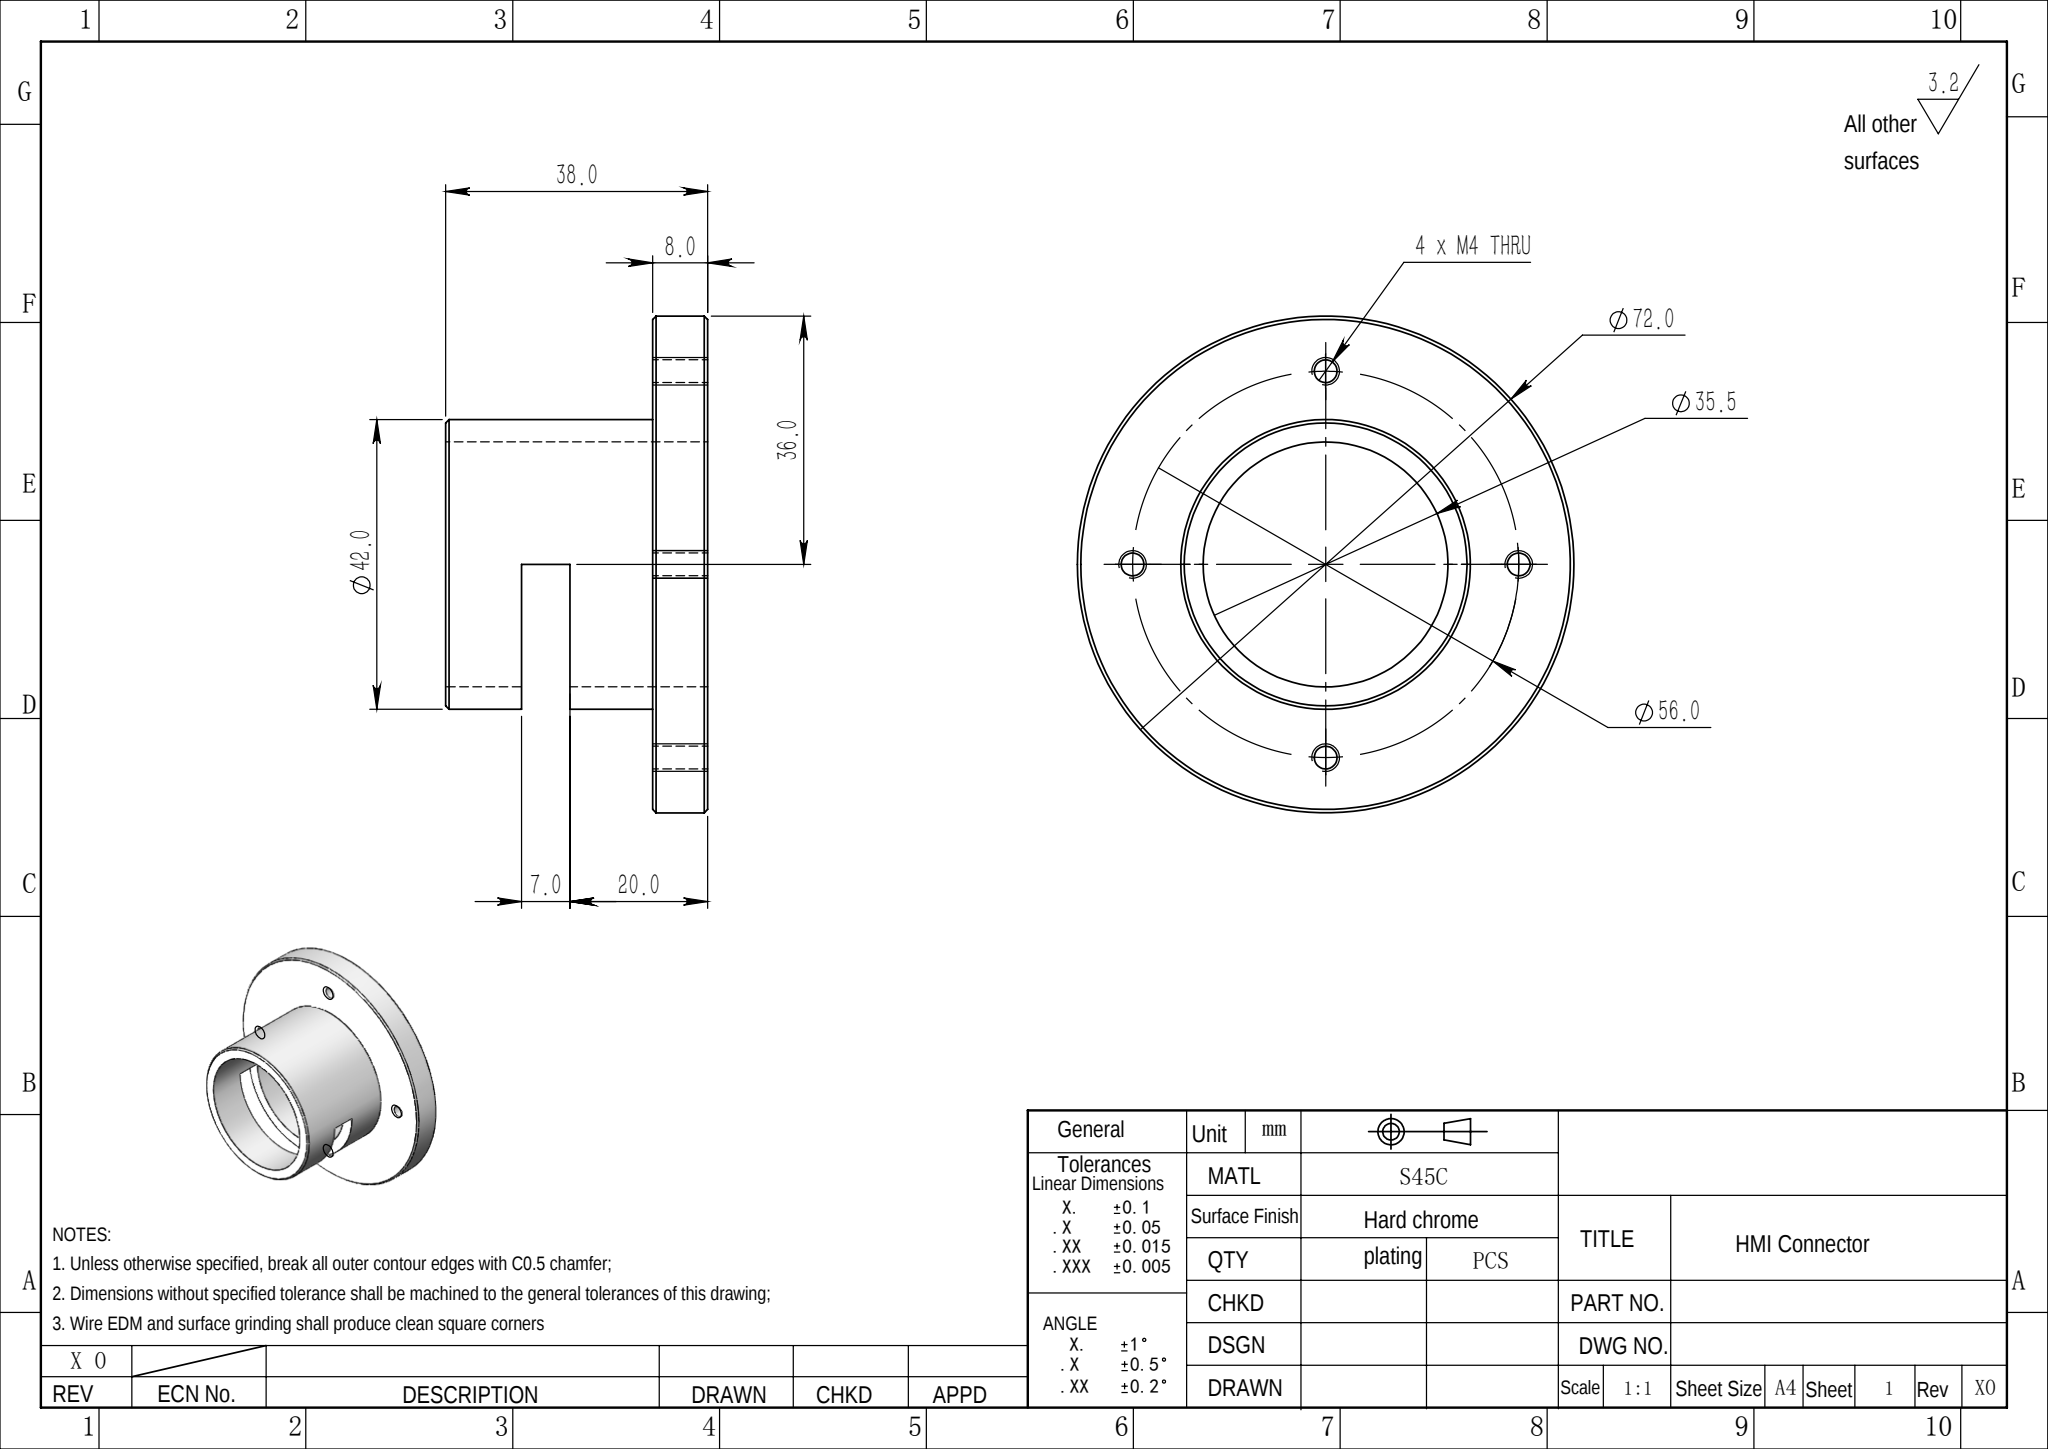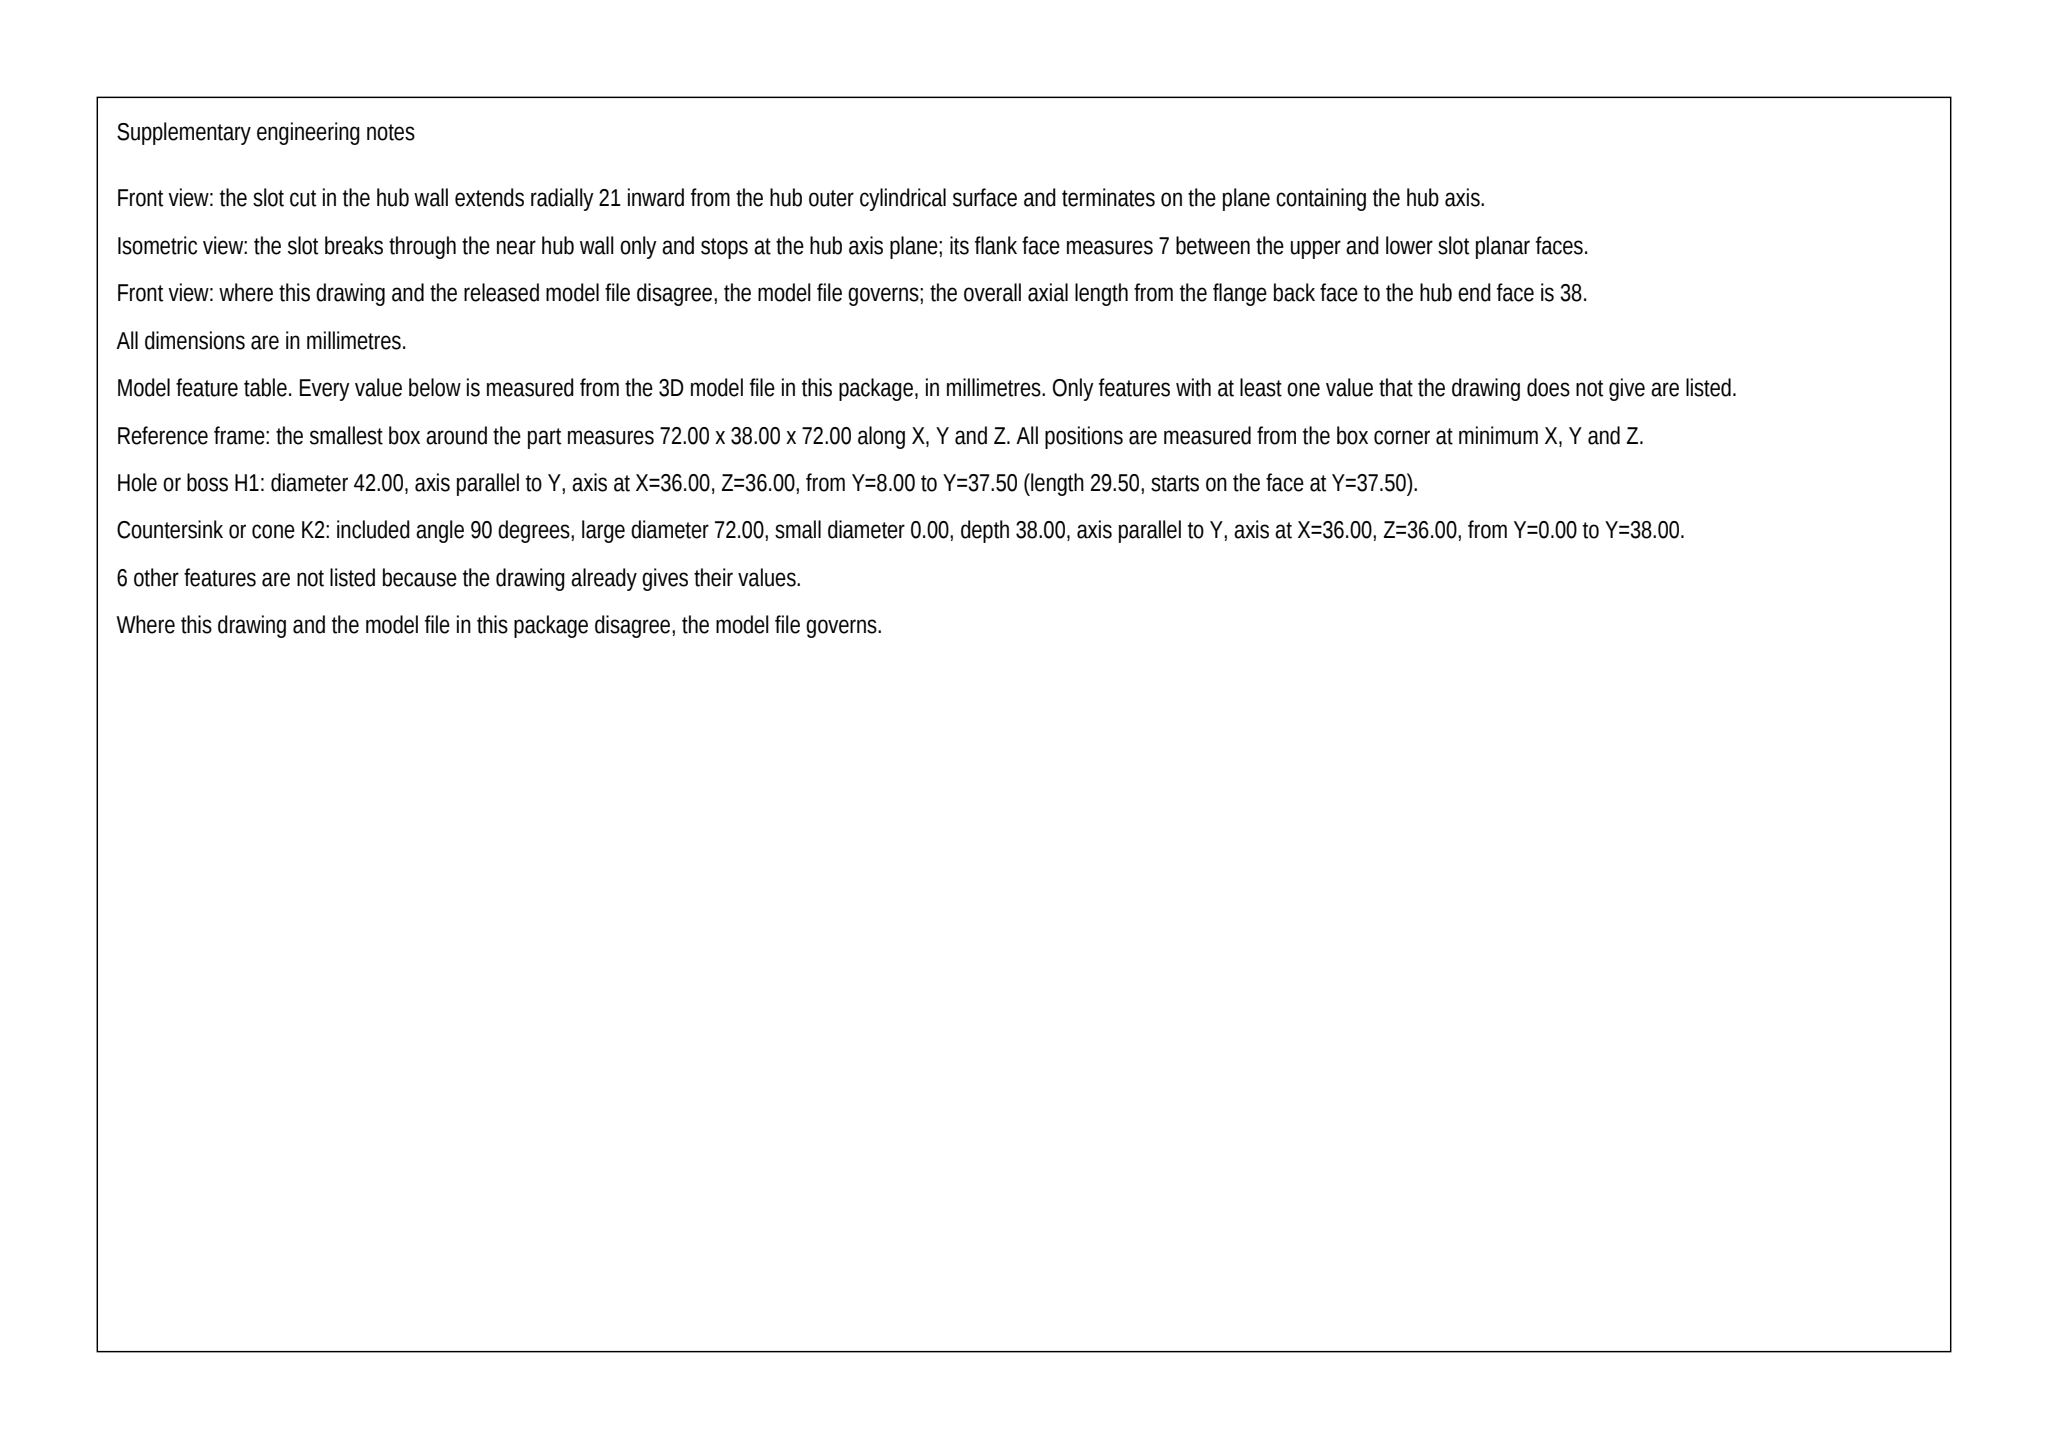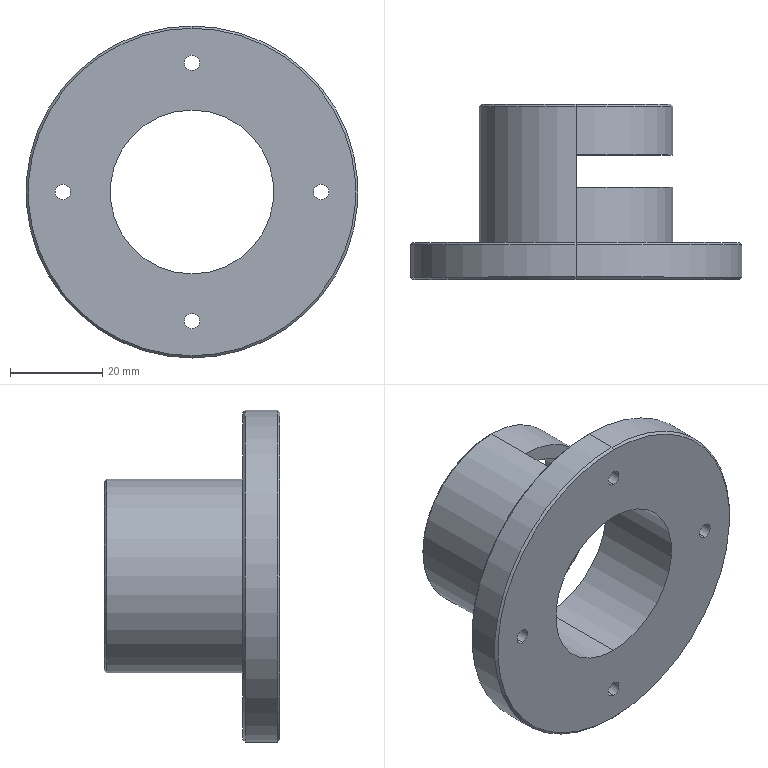Part | SolidWorks | mm | material S45C | 1 solid | 29 faces | box 72 x 38 x 72 mm | volume 34792 mm3 | cylinder 16 | plane 7 | cone 6 | commonest cylinder face diameters 3.3 x8 35.5 x3 42 x3 72 x2
build123d program:
from build123d import *

# Parameters (mm, degrees)
SKETCH1_R           = 36
BOSS_EXTRUDE1_DEPTH = 8
SKETCH2_R           = 21
BOSS_EXTRUDE2_DEPTH = 30
SKETCH3_R           = 17.75
CUT_EXTRUDE1_DEPTH  = 64.53
M4_TAPPED_HOLE1_D   = 3.3
CIRPATTERN1_COUNT   = 4
CHAMFER1_SIZE       = 0.5
CUT_EXTRUDE2_START  = -21
SKETCH6_W           = 45
SKETCH6_H           = 7
CUT_EXTRUDE2_DEPTH  = 21


with BuildPart() as part:
    # Sketch1 → Boss-Extrude1 (new body)
    with BuildSketch(Plane(origin=(0, 0, 0), x_dir=(1, 0, 0), z_dir=(0, 1, 0))):
        with Locations(Location((0, 0, 0), (0, 0, 270))):
            Circle(SKETCH1_R)
    extrude(amount=-BOSS_EXTRUDE1_DEPTH)

    # Sketch2 → Boss-Extrude2 (add)
    with BuildSketch(Plane(origin=(0, 0, 0), x_dir=(1, 0, 0), z_dir=(0, 1, 0))):
        with Locations(Location((0, 0, 0), (0, 0, 270))):
            Circle(SKETCH2_R)
    extrude(amount=BOSS_EXTRUDE2_DEPTH)

    # Sketch3 → Cut-Extrude1 (cut, through all)
    with BuildSketch(Plane(origin=(0, 30, 0), x_dir=(1, 0, 0), z_dir=(0, 1, 0))):
        with Locations(Location((0, 0, 0), (0, 0, 270))):
            Circle(SKETCH3_R)
    extrude(amount=-CUT_EXTRUDE1_DEPTH, mode=Mode.SUBTRACT)

    # M4 Tapped Hole1 (through all)
    with Locations(Plane(origin=(0, 0, 0), x_dir=(1, 0, 0), z_dir=(0, 1, 0))):
        with Locations((0, 28)):
            m4_tapped_hole1 = Hole(M4_TAPPED_HOLE1_D / 2)

    # CirPattern1: M4 Tapped Hole1 ×4 about axis
    cirpattern1_axis = Axis((0, 0, 0), (0, 1, 0))
    for i in range(1, CIRPATTERN1_COUNT):
        add(m4_tapped_hole1.rotate(cirpattern1_axis, i * 360 / CIRPATTERN1_COUNT), mode=Mode.SUBTRACT)

    # Chamfer1
    chamfer1_edges = [part.edges().sort_by_distance(p)[0] for p in [
        (0, 0, -36),
        (0, -8, -36),
        (0, 30, -21),
    ]]
    chamfer(chamfer1_edges, length=CHAMFER1_SIZE)

    # Sketch6 → Cut-Extrude2 (cut)
    with BuildSketch(Plane(origin=(21, 0, 0), x_dir=(0, 0, -1), z_dir=(1, 0, 0)).offset(CUT_EXTRUDE2_START)):
        with Locations((0, 15.5)):
            Rectangle(SKETCH6_W, SKETCH6_H)
    extrude(amount=CUT_EXTRUDE2_DEPTH, mode=Mode.SUBTRACT)


solid = part.part
STEP:
#1=CARTESIAN_POINT('',(0.,0.,35.5));
#2=VERTEX_POINT('',#1);
#3=CARTESIAN_POINT('',(0.,0.,-35.5));
#4=VERTEX_POINT('',#3);
#5=CARTESIAN_POINT('',(0.,0.,0.));
#6=DIRECTION('',(0.,1.,0.));
#7=DIRECTION('',(0.,0.,1.));
#8=AXIS2_PLACEMENT_3D('',#5,#6,#7);
#9=CIRCLE('',#8,35.5);
#10=EDGE_CURVE('',#2,#4,#9,.T.);
#11=ORIENTED_EDGE('',*,*,#10,.F.);
#12=CARTESIAN_POINT('',(0.,-0.5,36.));
#13=VERTEX_POINT('',#12);
#14=CARTESIAN_POINT('',(0.,0.,35.5));
#15=DIRECTION('',(0.,-0.7071,0.7071));
#16=VECTOR('',#15,1000.);
#17=LINE('',#14,#16);
#18=EDGE_CURVE('',#2,#13,#17,.T.);
#19=ORIENTED_EDGE('',*,*,#18,.T.);
#20=CARTESIAN_POINT('',(0.,-0.5,-36.));
#21=VERTEX_POINT('',#20);
#22=CARTESIAN_POINT('',(0.,-0.5,0.));
#23=DIRECTION('',(0.,-1.,0.));
#24=DIRECTION('',(0.,0.,1.));
#25=AXIS2_PLACEMENT_3D('',#22,#23,#24);
#26=CIRCLE('',#25,36.);
#27=EDGE_CURVE('',#21,#13,#26,.T.);
#28=ORIENTED_EDGE('',*,*,#27,.F.);
#29=CARTESIAN_POINT('',(0.,0.,-35.5));
#30=DIRECTION('',(0.,-0.7071,-0.7071));
#31=VECTOR('',#30,1000.);
#32=LINE('',#29,#31);
#33=EDGE_CURVE('',#4,#21,#32,.T.);
#34=ORIENTED_EDGE('',*,*,#33,.F.);
#35=EDGE_LOOP('',(#11,#19,#28,#34));
#36=FACE_OUTER_BOUND('',#35,.T.);
#37=CARTESIAN_POINT('',(0.,0.,0.));
#38=DIRECTION('',(0.,-1.,0.));
#39=DIRECTION('',(0.,0.,-1.));
#40=AXIS2_PLACEMENT_3D('',#37,#38,#39);
#41=CONICAL_SURFACE('',#40,35.5,0.7854);
#42=ADVANCED_FACE('',(#36),#41,.T.);
#43=CARTESIAN_POINT('',(0.,-8.,-35.5));
#44=VERTEX_POINT('',#43);
#45=CARTESIAN_POINT('',(0.,-8.,35.5));
#46=VERTEX_POINT('',#45);
#47=CARTESIAN_POINT('',(0.,-8.,0.));
#48=DIRECTION('',(0.,-1.,0.));
#49=DIRECTION('',(0.,0.,1.));
#50=AXIS2_PLACEMENT_3D('',#47,#48,#49);
#51=CIRCLE('',#50,35.5);
#52=EDGE_CURVE('',#44,#46,#51,.T.);
#53=ORIENTED_EDGE('',*,*,#52,.F.);
#54=CARTESIAN_POINT('',(0.,-7.5,-36.));
#55=VERTEX_POINT('',#54);
#56=CARTESIAN_POINT('',(0.,-7.5,-36.));
#57=DIRECTION('',(0.,0.7071,-0.7071));
#58=VECTOR('',#57,1000.);
#59=LINE('',#56,#58);
#60=EDGE_CURVE('',#44,#55,#59,.T.);
#61=ORIENTED_EDGE('',*,*,#60,.T.);
#62=CARTESIAN_POINT('',(0.,-7.5,36.));
#63=VERTEX_POINT('',#62);
#64=CARTESIAN_POINT('',(0.,-7.5,0.));
#65=DIRECTION('',(0.,1.,0.));
#66=DIRECTION('',(0.,0.,1.));
#67=AXIS2_PLACEMENT_3D('',#64,#65,#66);
#68=CIRCLE('',#67,36.);
#69=EDGE_CURVE('',#63,#55,#68,.T.);
#70=ORIENTED_EDGE('',*,*,#69,.F.);
#71=CARTESIAN_POINT('',(0.,-7.5,36.));
#72=DIRECTION('',(0.,0.7071,0.7071));
#73=VECTOR('',#72,1000.);
#74=LINE('',#71,#73);
#75=EDGE_CURVE('',#46,#63,#74,.T.);
#76=ORIENTED_EDGE('',*,*,#75,.F.);
#77=EDGE_LOOP('',(#53,#61,#70,#76));
#78=FACE_OUTER_BOUND('',#77,.T.);
#79=CARTESIAN_POINT('',(0.,-7.5,0.));
#80=DIRECTION('',(0.,1.,0.));
#81=DIRECTION('',(0.,0.,1.));
#82=AXIS2_PLACEMENT_3D('',#79,#80,#81);
#83=CONICAL_SURFACE('',#82,36.,0.7854);
#84=ADVANCED_FACE('',(#78),#83,.T.);
#85=CARTESIAN_POINT('',(0.,30.,20.5));
#86=VERTEX_POINT('',#85);
#87=CARTESIAN_POINT('',(0.,30.,-20.5));
#88=VERTEX_POINT('',#87);
#89=CARTESIAN_POINT('',(0.,30.,0.));
#90=DIRECTION('',(0.,1.,0.));
#91=DIRECTION('',(0.,0.,1.));
#92=AXIS2_PLACEMENT_3D('',#89,#90,#91);
#93=CIRCLE('',#92,20.5);
#94=EDGE_CURVE('',#86,#88,#93,.T.);
#95=ORIENTED_EDGE('',*,*,#94,.F.);
#96=CARTESIAN_POINT('',(0.,29.5,21.));
#97=VERTEX_POINT('',#96);
#98=CARTESIAN_POINT('',(0.,30.,20.5));
#99=DIRECTION('',(0.,-0.7071,0.7071));
#100=VECTOR('',#99,1000.);
#101=LINE('',#98,#100);
#102=EDGE_CURVE('',#86,#97,#101,.T.);
#103=ORIENTED_EDGE('',*,*,#102,.T.);
#104=CARTESIAN_POINT('',(0.,29.5,-21.));
#105=VERTEX_POINT('',#104);
#106=CARTESIAN_POINT('',(0.,29.5,0.));
#107=DIRECTION('',(0.,-1.,0.));
#108=DIRECTION('',(0.,0.,1.));
#109=AXIS2_PLACEMENT_3D('',#106,#107,#108);
#110=CIRCLE('',#109,21.);
#111=EDGE_CURVE('',#105,#97,#110,.T.);
#112=ORIENTED_EDGE('',*,*,#111,.F.);
#113=CARTESIAN_POINT('',(0.,30.,-20.5));
#114=DIRECTION('',(0.,-0.7071,-0.7071));
#115=VECTOR('',#114,1000.);
#116=LINE('',#113,#115);
#117=EDGE_CURVE('',#88,#105,#116,.T.);
#118=ORIENTED_EDGE('',*,*,#117,.F.);
#119=EDGE_LOOP('',(#95,#103,#112,#118));
#120=FACE_OUTER_BOUND('',#119,.T.);
#121=CARTESIAN_POINT('',(0.,30.,0.));
#122=DIRECTION('',(0.,-1.,0.));
#123=DIRECTION('',(0.,0.,-1.));
#124=AXIS2_PLACEMENT_3D('',#121,#122,#123);
#125=CONICAL_SURFACE('',#124,20.5,0.7854);
#126=ADVANCED_FACE('',(#120),#125,.T.);
#127=CARTESIAN_POINT('',(28.,-8.,-1.65));
#128=VERTEX_POINT('',#127);
#129=CARTESIAN_POINT('',(28.,-8.,1.65));
#130=VERTEX_POINT('',#129);
#131=CARTESIAN_POINT('',(28.,-8.,-0.));
#132=DIRECTION('',(0.,1.,0.));
#133=DIRECTION('',(0.,0.,1.));
#134=AXIS2_PLACEMENT_3D('',#131,#132,#133);
#135=CIRCLE('',#134,1.65);
#136=EDGE_CURVE('',#128,#130,#135,.T.);
#137=ORIENTED_EDGE('',*,*,#136,.F.);
#138=CARTESIAN_POINT('',(28.,0.,-1.65));
#139=VERTEX_POINT('',#138);
#140=CARTESIAN_POINT('',(28.,0.,-1.65));
#141=DIRECTION('',(0.,1.,0.));
#142=VECTOR('',#141,1000.);
#143=LINE('',#140,#142);
#144=EDGE_CURVE('',#128,#139,#143,.T.);
#145=ORIENTED_EDGE('',*,*,#144,.T.);
#146=CARTESIAN_POINT('',(28.,0.,1.65));
#147=VERTEX_POINT('',#146);
#148=CARTESIAN_POINT('',(28.,0.,-0.));
#149=DIRECTION('',(0.,1.,0.));
#150=DIRECTION('',(0.,0.,1.));
#151=AXIS2_PLACEMENT_3D('',#148,#149,#150);
#152=CIRCLE('',#151,1.65);
#153=EDGE_CURVE('',#139,#147,#152,.T.);
#154=ORIENTED_EDGE('',*,*,#153,.T.);
#155=CARTESIAN_POINT('',(28.,0.,1.65));
#156=DIRECTION('',(0.,1.,0.));
#157=VECTOR('',#156,1000.);
#158=LINE('',#155,#157);
#159=EDGE_CURVE('',#130,#147,#158,.T.);
#160=ORIENTED_EDGE('',*,*,#159,.F.);
#161=EDGE_LOOP('',(#137,#145,#154,#160));
#162=FACE_OUTER_BOUND('',#161,.T.);
#163=CARTESIAN_POINT('',(28.,0.,-0.));
#164=DIRECTION('',(0.,1.,0.));
#165=DIRECTION('',(0.,0.,1.));
#166=AXIS2_PLACEMENT_3D('',#163,#164,#165);
#167=CYLINDRICAL_SURFACE('',#166,1.65);
#168=ADVANCED_FACE('',(#162),#167,.F.);
#169=CARTESIAN_POINT('',(0.,-8.,26.35));
#170=VERTEX_POINT('',#169);
#171=CARTESIAN_POINT('',(0.,-8.,29.65));
#172=VERTEX_POINT('',#171);
#173=CARTESIAN_POINT('',(0.,-8.,28.));
#174=DIRECTION('',(0.,1.,0.));
#175=DIRECTION('',(0.,0.,1.));
#176=AXIS2_PLACEMENT_3D('',#173,#174,#175);
#177=CIRCLE('',#176,1.65);
#178=EDGE_CURVE('',#170,#172,#177,.T.);
#179=ORIENTED_EDGE('',*,*,#178,.F.);
#180=CARTESIAN_POINT('',(0.,0.,26.35));
#181=VERTEX_POINT('',#180);
#182=CARTESIAN_POINT('',(0.,0.,26.35));
#183=DIRECTION('',(0.,1.,0.));
#184=VECTOR('',#183,1000.);
#185=LINE('',#182,#184);
#186=EDGE_CURVE('',#170,#181,#185,.T.);
#187=ORIENTED_EDGE('',*,*,#186,.T.);
#188=CARTESIAN_POINT('',(0.,0.,29.65));
#189=VERTEX_POINT('',#188);
#190=CARTESIAN_POINT('',(0.,0.,28.));
#191=DIRECTION('',(0.,1.,0.));
#192=DIRECTION('',(0.,0.,1.));
#193=AXIS2_PLACEMENT_3D('',#190,#191,#192);
#194=CIRCLE('',#193,1.65);
#195=EDGE_CURVE('',#181,#189,#194,.T.);
#196=ORIENTED_EDGE('',*,*,#195,.T.);
#197=CARTESIAN_POINT('',(0.,0.,29.65));
#198=DIRECTION('',(0.,1.,0.));
#199=VECTOR('',#198,1000.);
#200=LINE('',#197,#199);
#201=EDGE_CURVE('',#172,#189,#200,.T.);
#202=ORIENTED_EDGE('',*,*,#201,.F.);
#203=EDGE_LOOP('',(#179,#187,#196,#202));
#204=FACE_OUTER_BOUND('',#203,.T.);
#205=CARTESIAN_POINT('',(0.,0.,28.));
#206=DIRECTION('',(0.,1.,0.));
#207=DIRECTION('',(0.,0.,1.));
#208=AXIS2_PLACEMENT_3D('',#205,#206,#207);
#209=CYLINDRICAL_SURFACE('',#208,1.65);
#210=ADVANCED_FACE('',(#204),#209,.F.);
#211=CARTESIAN_POINT('',(-28.,-8.,-1.65));
#212=VERTEX_POINT('',#211);
#213=CARTESIAN_POINT('',(-28.,-8.,1.65));
#214=VERTEX_POINT('',#213);
#215=CARTESIAN_POINT('',(-28.,-8.,0.));
#216=DIRECTION('',(0.,1.,0.));
#217=DIRECTION('',(0.,0.,1.));
#218=AXIS2_PLACEMENT_3D('',#215,#216,#217);
#219=CIRCLE('',#218,1.65);
#220=EDGE_CURVE('',#212,#214,#219,.T.);
#221=ORIENTED_EDGE('',*,*,#220,.F.);
#222=CARTESIAN_POINT('',(-28.,0.,-1.65));
#223=VERTEX_POINT('',#222);
#224=CARTESIAN_POINT('',(-28.,0.,-1.65));
#225=DIRECTION('',(0.,1.,0.));
#226=VECTOR('',#225,1000.);
#227=LINE('',#224,#226);
#228=EDGE_CURVE('',#212,#223,#227,.T.);
#229=ORIENTED_EDGE('',*,*,#228,.T.);
#230=CARTESIAN_POINT('',(-28.,0.,1.65));
#231=VERTEX_POINT('',#230);
#232=CARTESIAN_POINT('',(-28.,0.,0.));
#233=DIRECTION('',(0.,1.,0.));
#234=DIRECTION('',(0.,0.,1.));
#235=AXIS2_PLACEMENT_3D('',#232,#233,#234);
#236=CIRCLE('',#235,1.65);
#237=EDGE_CURVE('',#223,#231,#236,.T.);
#238=ORIENTED_EDGE('',*,*,#237,.T.);
#239=CARTESIAN_POINT('',(-28.,0.,1.65));
#240=DIRECTION('',(0.,1.,0.));
#241=VECTOR('',#240,1000.);
#242=LINE('',#239,#241);
#243=EDGE_CURVE('',#214,#231,#242,.T.);
#244=ORIENTED_EDGE('',*,*,#243,.F.);
#245=EDGE_LOOP('',(#221,#229,#238,#244));
#246=FACE_OUTER_BOUND('',#245,.T.);
#247=CARTESIAN_POINT('',(-28.,0.,0.));
#248=DIRECTION('',(0.,1.,0.));
#249=DIRECTION('',(0.,0.,1.));
#250=AXIS2_PLACEMENT_3D('',#247,#248,#249);
#251=CYLINDRICAL_SURFACE('',#250,1.65);
#252=ADVANCED_FACE('',(#246),#251,.F.);
#253=CARTESIAN_POINT('',(0.,-8.,-29.65));
#254=VERTEX_POINT('',#253);
#255=CARTESIAN_POINT('',(0.,-8.,-26.35));
#256=VERTEX_POINT('',#255);
#257=CARTESIAN_POINT('',(0.,-8.,-28.));
#258=DIRECTION('',(0.,1.,0.));
#259=DIRECTION('',(0.,0.,1.));
#260=AXIS2_PLACEMENT_3D('',#257,#258,#259);
#261=CIRCLE('',#260,1.65);
#262=EDGE_CURVE('',#254,#256,#261,.T.);
#263=ORIENTED_EDGE('',*,*,#262,.F.);
#264=CARTESIAN_POINT('',(0.,0.,-29.65));
#265=VERTEX_POINT('',#264);
#266=CARTESIAN_POINT('',(0.,0.,-29.65));
#267=DIRECTION('',(0.,1.,0.));
#268=VECTOR('',#267,1000.);
#269=LINE('',#266,#268);
#270=EDGE_CURVE('',#254,#265,#269,.T.);
#271=ORIENTED_EDGE('',*,*,#270,.T.);
#272=CARTESIAN_POINT('',(0.,0.,-26.35));
#273=VERTEX_POINT('',#272);
#274=CARTESIAN_POINT('',(0.,0.,-28.));
#275=DIRECTION('',(0.,1.,0.));
#276=DIRECTION('',(0.,0.,1.));
#277=AXIS2_PLACEMENT_3D('',#274,#275,#276);
#278=CIRCLE('',#277,1.65);
#279=EDGE_CURVE('',#265,#273,#278,.T.);
#280=ORIENTED_EDGE('',*,*,#279,.T.);
#281=CARTESIAN_POINT('',(0.,0.,-26.35));
#282=DIRECTION('',(0.,1.,0.));
#283=VECTOR('',#282,1000.);
#284=LINE('',#281,#283);
#285=EDGE_CURVE('',#256,#273,#284,.T.);
#286=ORIENTED_EDGE('',*,*,#285,.F.);
#287=EDGE_LOOP('',(#263,#271,#280,#286));
#288=FACE_OUTER_BOUND('',#287,.T.);
#289=CARTESIAN_POINT('',(0.,0.,-28.));
#290=DIRECTION('',(0.,1.,0.));
#291=DIRECTION('',(0.,0.,1.));
#292=AXIS2_PLACEMENT_3D('',#289,#290,#291);
#293=CYLINDRICAL_SURFACE('',#292,1.65);
#294=ADVANCED_FACE('',(#288),#293,.F.);
#295=ORIENTED_EDGE('',*,*,#69,.T.);
#296=CARTESIAN_POINT('',(0.,-8.,-36.));
#297=DIRECTION('',(0.,1.,0.));
#298=VECTOR('',#297,1000.);
#299=LINE('',#296,#298);
#300=EDGE_CURVE('',#55,#21,#299,.T.);
#301=ORIENTED_EDGE('',*,*,#300,.T.);
#302=ORIENTED_EDGE('',*,*,#27,.T.);
#303=CARTESIAN_POINT('',(0.,-8.,36.));
#304=DIRECTION('',(0.,1.,0.));
#305=VECTOR('',#304,1000.);
#306=LINE('',#303,#305);
#307=EDGE_CURVE('',#63,#13,#306,.T.);
#308=ORIENTED_EDGE('',*,*,#307,.F.);
#309=EDGE_LOOP('',(#295,#301,#302,#308));
#310=FACE_OUTER_BOUND('',#309,.T.);
#311=CARTESIAN_POINT('',(0.,-8.,0.));
#312=DIRECTION('',(0.,1.,0.));
#313=DIRECTION('',(0.,0.,1.));
#314=AXIS2_PLACEMENT_3D('',#311,#312,#313);
#315=CYLINDRICAL_SURFACE('',#314,36.);
#316=ADVANCED_FACE('',(#310),#315,.T.);
#317=CARTESIAN_POINT('',(0.,-8.,-17.75));
#318=VERTEX_POINT('',#317);
#319=CARTESIAN_POINT('',(0.,-8.,17.75));
#320=VERTEX_POINT('',#319);
#321=CARTESIAN_POINT('',(0.,-8.,0.));
#322=DIRECTION('',(0.,1.,0.));
#323=DIRECTION('',(0.,0.,1.));
#324=AXIS2_PLACEMENT_3D('',#321,#322,#323);
#325=CIRCLE('',#324,17.75);
#326=EDGE_CURVE('',#318,#320,#325,.T.);
#327=ORIENTED_EDGE('',*,*,#326,.F.);
#328=CARTESIAN_POINT('',(0.,12.,-17.75));
#329=VERTEX_POINT('',#328);
#330=CARTESIAN_POINT('',(0.,-8.,-17.75));
#331=DIRECTION('',(0.,1.,0.));
#332=VECTOR('',#331,1000.);
#333=LINE('',#330,#332);
#334=EDGE_CURVE('',#318,#329,#333,.T.);
#335=ORIENTED_EDGE('',*,*,#334,.T.);
#336=CARTESIAN_POINT('',(0.,19.,-17.75));
#337=VERTEX_POINT('',#336);
#338=CARTESIAN_POINT('',(0.,-8.,-17.75));
#339=DIRECTION('',(0.,-1.,0.));
#340=VECTOR('',#339,1000.);
#341=LINE('',#338,#340);
#342=EDGE_CURVE('',#337,#329,#341,.T.);
#343=ORIENTED_EDGE('',*,*,#342,.F.);
#344=CARTESIAN_POINT('',(0.,30.,-17.75));
#345=VERTEX_POINT('',#344);
#346=CARTESIAN_POINT('',(0.,-8.,-17.75));
#347=DIRECTION('',(0.,1.,0.));
#348=VECTOR('',#347,1000.);
#349=LINE('',#346,#348);
#350=EDGE_CURVE('',#337,#345,#349,.T.);
#351=ORIENTED_EDGE('',*,*,#350,.T.);
#352=CARTESIAN_POINT('',(0.,30.,17.75));
#353=VERTEX_POINT('',#352);
#354=CARTESIAN_POINT('',(0.,30.,0.));
#355=DIRECTION('',(0.,1.,0.));
#356=DIRECTION('',(0.,0.,1.));
#357=AXIS2_PLACEMENT_3D('',#354,#355,#356);
#358=CIRCLE('',#357,17.75);
#359=EDGE_CURVE('',#345,#353,#358,.T.);
#360=ORIENTED_EDGE('',*,*,#359,.T.);
#361=CARTESIAN_POINT('',(0.,19.,17.75));
#362=VERTEX_POINT('',#361);
#363=CARTESIAN_POINT('',(0.,-8.,17.75));
#364=DIRECTION('',(0.,1.,0.));
#365=VECTOR('',#364,1000.);
#366=LINE('',#363,#365);
#367=EDGE_CURVE('',#362,#353,#366,.T.);
#368=ORIENTED_EDGE('',*,*,#367,.F.);
#369=CARTESIAN_POINT('',(0.,12.,17.75));
#370=VERTEX_POINT('',#369);
#371=CARTESIAN_POINT('',(0.,-8.,17.75));
#372=DIRECTION('',(0.,1.,0.));
#373=VECTOR('',#372,1000.);
#374=LINE('',#371,#373);
#375=EDGE_CURVE('',#370,#362,#374,.T.);
#376=ORIENTED_EDGE('',*,*,#375,.F.);
#377=CARTESIAN_POINT('',(0.,-8.,17.75));
#378=DIRECTION('',(0.,1.,0.));
#379=VECTOR('',#378,1000.);
#380=LINE('',#377,#379);
#381=EDGE_CURVE('',#320,#370,#380,.T.);
#382=ORIENTED_EDGE('',*,*,#381,.F.);
#383=EDGE_LOOP('',(#327,#335,#343,#351,#360,#368,#376,#382));
#384=FACE_OUTER_BOUND('',#383,.T.);
#385=CARTESIAN_POINT('',(0.,-8.,0.));
#386=DIRECTION('',(0.,1.,0.));
#387=DIRECTION('',(0.,0.,1.));
#388=AXIS2_PLACEMENT_3D('',#385,#386,#387);
#389=CYLINDRICAL_SURFACE('',#388,17.75);
#390=ADVANCED_FACE('',(#384),#389,.F.);
#391=ORIENTED_EDGE('',*,*,#334,.F.);
#392=CARTESIAN_POINT('',(0.,-8.,0.));
#393=DIRECTION('',(0.,1.,0.));
#394=DIRECTION('',(0.,0.,1.));
#395=AXIS2_PLACEMENT_3D('',#392,#393,#394);
#396=CIRCLE('',#395,17.75);
#397=EDGE_CURVE('',#320,#318,#396,.T.);
#398=ORIENTED_EDGE('',*,*,#397,.F.);
#399=ORIENTED_EDGE('',*,*,#381,.T.);
#400=CARTESIAN_POINT('',(0.,12.,0.));
#401=DIRECTION('',(0.,1.,0.));
#402=DIRECTION('',(0.,0.,-1.));
#403=AXIS2_PLACEMENT_3D('',#400,#401,#402);
#404=CIRCLE('',#403,17.75);
#405=EDGE_CURVE('',#370,#329,#404,.T.);
#406=ORIENTED_EDGE('',*,*,#405,.T.);
#407=EDGE_LOOP('',(#391,#398,#399,#406));
#408=FACE_OUTER_BOUND('',#407,.T.);
#409=CARTESIAN_POINT('',(0.,-8.,0.));
#410=DIRECTION('',(0.,1.,0.));
#411=DIRECTION('',(0.,0.,1.));
#412=AXIS2_PLACEMENT_3D('',#409,#410,#411);
#413=CYLINDRICAL_SURFACE('',#412,17.75);
#414=ADVANCED_FACE('',(#408),#413,.F.);
#415=ORIENTED_EDGE('',*,*,#111,.T.);
#416=CARTESIAN_POINT('',(0.,19.,21.));
#417=VERTEX_POINT('',#416);
#418=CARTESIAN_POINT('',(0.,30.,21.));
#419=DIRECTION('',(0.,-1.,0.));
#420=VECTOR('',#419,1000.);
#421=LINE('',#418,#420);
#422=EDGE_CURVE('',#97,#417,#421,.T.);
#423=ORIENTED_EDGE('',*,*,#422,.T.);
#424=CARTESIAN_POINT('',(0.,19.,-21.));
#425=VERTEX_POINT('',#424);
#426=CARTESIAN_POINT('',(0.,19.,0.));
#427=DIRECTION('',(0.,1.,0.));
#428=DIRECTION('',(0.,0.,1.));
#429=AXIS2_PLACEMENT_3D('',#426,#427,#428);
#430=CIRCLE('',#429,21.);
#431=EDGE_CURVE('',#417,#425,#430,.T.);
#432=ORIENTED_EDGE('',*,*,#431,.T.);
#433=CARTESIAN_POINT('',(0.,30.,-21.));
#434=DIRECTION('',(0.,-1.,0.));
#435=VECTOR('',#434,1000.);
#436=LINE('',#433,#435);
#437=EDGE_CURVE('',#105,#425,#436,.T.);
#438=ORIENTED_EDGE('',*,*,#437,.F.);
#439=EDGE_LOOP('',(#415,#423,#432,#438));
#440=FACE_OUTER_BOUND('',#439,.T.);
#441=CARTESIAN_POINT('',(0.,30.,0.));
#442=DIRECTION('',(0.,-1.,0.));
#443=DIRECTION('',(0.,0.,-1.));
#444=AXIS2_PLACEMENT_3D('',#441,#442,#443);
#445=CYLINDRICAL_SURFACE('',#444,21.);
#446=ADVANCED_FACE('',(#440),#445,.T.);
#447=CARTESIAN_POINT('',(0.,12.,-21.));
#448=VERTEX_POINT('',#447);
#449=CARTESIAN_POINT('',(0.,12.,21.));
#450=VERTEX_POINT('',#449);
#451=CARTESIAN_POINT('',(0.,12.,0.));
#452=DIRECTION('',(0.,-1.,-0.));
#453=DIRECTION('',(0.,0.,-1.));
#454=AXIS2_PLACEMENT_3D('',#451,#452,#453);
#455=CIRCLE('',#454,21.);
#456=EDGE_CURVE('',#448,#450,#455,.T.);
#457=ORIENTED_EDGE('',*,*,#456,.T.);
#458=CARTESIAN_POINT('',(0.,0.,21.));
#459=VERTEX_POINT('',#458);
#460=CARTESIAN_POINT('',(0.,30.,21.));
#461=DIRECTION('',(0.,-1.,0.));
#462=VECTOR('',#461,1000.);
#463=LINE('',#460,#462);
#464=EDGE_CURVE('',#450,#459,#463,.T.);
#465=ORIENTED_EDGE('',*,*,#464,.T.);
#466=CARTESIAN_POINT('',(0.,0.,-21.));
#467=VERTEX_POINT('',#466);
#468=CARTESIAN_POINT('',(0.,0.,0.));
#469=DIRECTION('',(0.,1.,0.));
#470=DIRECTION('',(0.,0.,1.));
#471=AXIS2_PLACEMENT_3D('',#468,#469,#470);
#472=CIRCLE('',#471,21.);
#473=EDGE_CURVE('',#459,#467,#472,.T.);
#474=ORIENTED_EDGE('',*,*,#473,.T.);
#475=CARTESIAN_POINT('',(0.,30.,-21.));
#476=DIRECTION('',(0.,-1.,0.));
#477=VECTOR('',#476,1000.);
#478=LINE('',#475,#477);
#479=EDGE_CURVE('',#448,#467,#478,.T.);
#480=ORIENTED_EDGE('',*,*,#479,.F.);
#481=EDGE_LOOP('',(#457,#465,#474,#480));
#482=FACE_OUTER_BOUND('',#481,.T.);
#483=CARTESIAN_POINT('',(0.,30.,0.));
#484=DIRECTION('',(0.,-1.,0.));
#485=DIRECTION('',(0.,0.,-1.));
#486=AXIS2_PLACEMENT_3D('',#483,#484,#485);
#487=CYLINDRICAL_SURFACE('',#486,21.);
#488=ADVANCED_FACE('',(#482),#487,.T.);
#489=ORIENTED_EDGE('',*,*,#422,.F.);
#490=CARTESIAN_POINT('',(0.,29.5,0.));
#491=DIRECTION('',(0.,-1.,0.));
#492=DIRECTION('',(0.,0.,1.));
#493=AXIS2_PLACEMENT_3D('',#490,#491,#492);
#494=CIRCLE('',#493,21.);
#495=EDGE_CURVE('',#97,#105,#494,.T.);
#496=ORIENTED_EDGE('',*,*,#495,.T.);
#497=ORIENTED_EDGE('',*,*,#437,.T.);
#498=CARTESIAN_POINT('',(0.,30.,-21.));
#499=DIRECTION('',(0.,1.,0.));
#500=VECTOR('',#499,1000.);
#501=LINE('',#498,#500);
#502=EDGE_CURVE('',#448,#425,#501,.T.);
#503=ORIENTED_EDGE('',*,*,#502,.F.);
#504=ORIENTED_EDGE('',*,*,#479,.T.);
#505=CARTESIAN_POINT('',(0.,0.,0.));
#506=DIRECTION('',(0.,1.,0.));
#507=DIRECTION('',(0.,0.,1.));
#508=AXIS2_PLACEMENT_3D('',#505,#506,#507);
#509=CIRCLE('',#508,21.);
#510=EDGE_CURVE('',#467,#459,#509,.T.);
#511=ORIENTED_EDGE('',*,*,#510,.T.);
#512=ORIENTED_EDGE('',*,*,#464,.F.);
#513=CARTESIAN_POINT('',(0.,30.,21.));
#514=DIRECTION('',(0.,-1.,0.));
#515=VECTOR('',#514,1000.);
#516=LINE('',#513,#515);
#517=EDGE_CURVE('',#417,#450,#516,.T.);
#518=ORIENTED_EDGE('',*,*,#517,.F.);
#519=EDGE_LOOP('',(#489,#496,#497,#503,#504,#511,#512,#518));
#520=FACE_OUTER_BOUND('',#519,.T.);
#521=CARTESIAN_POINT('',(0.,30.,0.));
#522=DIRECTION('',(0.,-1.,0.));
#523=DIRECTION('',(0.,0.,-1.));
#524=AXIS2_PLACEMENT_3D('',#521,#522,#523);
#525=CYLINDRICAL_SURFACE('',#524,21.);
#526=ADVANCED_FACE('',(#520),#525,.T.);
#527=ORIENTED_EDGE('',*,*,#350,.F.);
#528=CARTESIAN_POINT('',(0.,19.,0.));
#529=DIRECTION('',(0.,-1.,0.));
#530=DIRECTION('',(0.,0.,1.));
#531=AXIS2_PLACEMENT_3D('',#528,#529,#530);
#532=CIRCLE('',#531,17.75);
#533=EDGE_CURVE('',#337,#362,#532,.T.);
#534=ORIENTED_EDGE('',*,*,#533,.T.);
#535=ORIENTED_EDGE('',*,*,#367,.T.);
#536=CARTESIAN_POINT('',(0.,30.,0.));
#537=DIRECTION('',(0.,1.,0.));
#538=DIRECTION('',(0.,0.,1.));
#539=AXIS2_PLACEMENT_3D('',#536,#537,#538);
#540=CIRCLE('',#539,17.75);
#541=EDGE_CURVE('',#353,#345,#540,.T.);
#542=ORIENTED_EDGE('',*,*,#541,.T.);
#543=EDGE_LOOP('',(#527,#534,#535,#542));
#544=FACE_OUTER_BOUND('',#543,.T.);
#545=CARTESIAN_POINT('',(0.,-8.,0.));
#546=DIRECTION('',(0.,1.,0.));
#547=DIRECTION('',(0.,0.,1.));
#548=AXIS2_PLACEMENT_3D('',#545,#546,#547);
#549=CYLINDRICAL_SURFACE('',#548,17.75);
#550=ADVANCED_FACE('',(#544),#549,.F.);
#551=ORIENTED_EDGE('',*,*,#300,.F.);
#552=CARTESIAN_POINT('',(0.,-7.5,0.));
#553=DIRECTION('',(0.,1.,0.));
#554=DIRECTION('',(0.,0.,1.));
#555=AXIS2_PLACEMENT_3D('',#552,#553,#554);
#556=CIRCLE('',#555,36.);
#557=EDGE_CURVE('',#55,#63,#556,.T.);
#558=ORIENTED_EDGE('',*,*,#557,.T.);
#559=ORIENTED_EDGE('',*,*,#307,.T.);
#560=CARTESIAN_POINT('',(0.,-0.5,0.));
#561=DIRECTION('',(0.,-1.,0.));
#562=DIRECTION('',(0.,0.,1.));
#563=AXIS2_PLACEMENT_3D('',#560,#561,#562);
#564=CIRCLE('',#563,36.);
#565=EDGE_CURVE('',#13,#21,#564,.T.);
#566=ORIENTED_EDGE('',*,*,#565,.T.);
#567=EDGE_LOOP('',(#551,#558,#559,#566));
#568=FACE_OUTER_BOUND('',#567,.T.);
#569=CARTESIAN_POINT('',(0.,-8.,0.));
#570=DIRECTION('',(0.,1.,0.));
#571=DIRECTION('',(0.,0.,1.));
#572=AXIS2_PLACEMENT_3D('',#569,#570,#571);
#573=CYLINDRICAL_SURFACE('',#572,36.);
#574=ADVANCED_FACE('',(#568),#573,.T.);
#575=CARTESIAN_POINT('',(0.,-8.,0.));
#576=DIRECTION('',(0.,-1.,0.));
#577=DIRECTION('',(0.,0.,1.));
#578=AXIS2_PLACEMENT_3D('',#575,#576,#577);
#579=CIRCLE('',#578,35.5);
#580=EDGE_CURVE('',#46,#44,#579,.T.);
#581=ORIENTED_EDGE('',*,*,#580,.T.);
#582=ORIENTED_EDGE('',*,*,#52,.T.);
#583=EDGE_LOOP('',(#581,#582));
#584=FACE_OUTER_BOUND('',#583,.T.);
#585=CARTESIAN_POINT('',(28.,-8.,-0.));
#586=DIRECTION('',(0.,1.,0.));
#587=DIRECTION('',(0.,0.,1.));
#588=AXIS2_PLACEMENT_3D('',#585,#586,#587);
#589=CIRCLE('',#588,1.65);
#590=EDGE_CURVE('',#130,#128,#589,.T.);
#591=ORIENTED_EDGE('',*,*,#590,.T.);
#592=ORIENTED_EDGE('',*,*,#136,.T.);
#593=EDGE_LOOP('',(#591,#592));
#594=FACE_BOUND('',#593,.T.);
#595=CARTESIAN_POINT('',(0.,-8.,28.));
#596=DIRECTION('',(0.,1.,0.));
#597=DIRECTION('',(0.,0.,1.));
#598=AXIS2_PLACEMENT_3D('',#595,#596,#597);
#599=CIRCLE('',#598,1.65);
#600=EDGE_CURVE('',#172,#170,#599,.T.);
#601=ORIENTED_EDGE('',*,*,#600,.T.);
#602=ORIENTED_EDGE('',*,*,#178,.T.);
#603=EDGE_LOOP('',(#601,#602));
#604=FACE_BOUND('',#603,.T.);
#605=CARTESIAN_POINT('',(-28.,-8.,0.));
#606=DIRECTION('',(0.,1.,0.));
#607=DIRECTION('',(0.,0.,1.));
#608=AXIS2_PLACEMENT_3D('',#605,#606,#607);
#609=CIRCLE('',#608,1.65);
#610=EDGE_CURVE('',#214,#212,#609,.T.);
#611=ORIENTED_EDGE('',*,*,#610,.T.);
#612=ORIENTED_EDGE('',*,*,#220,.T.);
#613=EDGE_LOOP('',(#611,#612));
#614=FACE_BOUND('',#613,.T.);
#615=CARTESIAN_POINT('',(0.,-8.,-28.));
#616=DIRECTION('',(0.,1.,0.));
#617=DIRECTION('',(0.,0.,1.));
#618=AXIS2_PLACEMENT_3D('',#615,#616,#617);
#619=CIRCLE('',#618,1.65);
#620=EDGE_CURVE('',#256,#254,#619,.T.);
#621=ORIENTED_EDGE('',*,*,#620,.T.);
#622=ORIENTED_EDGE('',*,*,#262,.T.);
#623=EDGE_LOOP('',(#621,#622));
#624=FACE_BOUND('',#623,.T.);
#625=ORIENTED_EDGE('',*,*,#397,.T.);
#626=ORIENTED_EDGE('',*,*,#326,.T.);
#627=EDGE_LOOP('',(#625,#626));
#628=FACE_BOUND('',#627,.T.);
#629=CARTESIAN_POINT('',(0.,-8.,0.));
#630=DIRECTION('',(0.,1.,0.));
#631=DIRECTION('',(0.,0.,1.));
#632=AXIS2_PLACEMENT_3D('',#629,#630,#631);
#633=PLANE('',#632);
#634=ADVANCED_FACE('',(#584,#594,#604,#614,#624,#628),#633,.F.);
#635=CARTESIAN_POINT('',(0.,0.,0.));
#636=DIRECTION('',(0.,1.,0.));
#637=DIRECTION('',(0.,0.,1.));
#638=AXIS2_PLACEMENT_3D('',#635,#636,#637);
#639=CIRCLE('',#638,35.5);
#640=EDGE_CURVE('',#4,#2,#639,.T.);
#641=ORIENTED_EDGE('',*,*,#640,.T.);
#642=ORIENTED_EDGE('',*,*,#10,.T.);
#643=EDGE_LOOP('',(#641,#642));
#644=FACE_OUTER_BOUND('',#643,.T.);
#645=CARTESIAN_POINT('',(28.,0.,-0.));
#646=DIRECTION('',(0.,1.,0.));
#647=DIRECTION('',(0.,0.,1.));
#648=AXIS2_PLACEMENT_3D('',#645,#646,#647);
#649=CIRCLE('',#648,1.65);
#650=EDGE_CURVE('',#147,#139,#649,.T.);
#651=ORIENTED_EDGE('',*,*,#650,.F.);
#652=ORIENTED_EDGE('',*,*,#153,.F.);
#653=EDGE_LOOP('',(#651,#652));
#654=FACE_BOUND('',#653,.T.);
#655=CARTESIAN_POINT('',(0.,0.,28.));
#656=DIRECTION('',(0.,1.,0.));
#657=DIRECTION('',(0.,0.,1.));
#658=AXIS2_PLACEMENT_3D('',#655,#656,#657);
#659=CIRCLE('',#658,1.65);
#660=EDGE_CURVE('',#189,#181,#659,.T.);
#661=ORIENTED_EDGE('',*,*,#660,.F.);
#662=ORIENTED_EDGE('',*,*,#195,.F.);
#663=EDGE_LOOP('',(#661,#662));
#664=FACE_BOUND('',#663,.T.);
#665=CARTESIAN_POINT('',(-28.,0.,0.));
#666=DIRECTION('',(0.,1.,0.));
#667=DIRECTION('',(0.,0.,1.));
#668=AXIS2_PLACEMENT_3D('',#665,#666,#667);
#669=CIRCLE('',#668,1.65);
#670=EDGE_CURVE('',#231,#223,#669,.T.);
#671=ORIENTED_EDGE('',*,*,#670,.F.);
#672=ORIENTED_EDGE('',*,*,#237,.F.);
#673=EDGE_LOOP('',(#671,#672));
#674=FACE_BOUND('',#673,.T.);
#675=CARTESIAN_POINT('',(0.,0.,-28.));
#676=DIRECTION('',(0.,1.,0.));
#677=DIRECTION('',(0.,0.,1.));
#678=AXIS2_PLACEMENT_3D('',#675,#676,#677);
#679=CIRCLE('',#678,1.65);
#680=EDGE_CURVE('',#273,#265,#679,.T.);
#681=ORIENTED_EDGE('',*,*,#680,.F.);
#682=ORIENTED_EDGE('',*,*,#279,.F.);
#683=EDGE_LOOP('',(#681,#682));
#684=FACE_BOUND('',#683,.T.);
#685=ORIENTED_EDGE('',*,*,#510,.F.);
#686=ORIENTED_EDGE('',*,*,#473,.F.);
#687=EDGE_LOOP('',(#685,#686));
#688=FACE_BOUND('',#687,.T.);
#689=CARTESIAN_POINT('',(0.,0.,0.));
#690=DIRECTION('',(0.,1.,0.));
#691=DIRECTION('',(0.,0.,1.));
#692=AXIS2_PLACEMENT_3D('',#689,#690,#691);
#693=PLANE('',#692);
#694=ADVANCED_FACE('',(#644,#654,#664,#674,#684,#688),#693,.T.);
#695=CARTESIAN_POINT('',(0.,30.,0.));
#696=DIRECTION('',(0.,1.,0.));
#697=DIRECTION('',(0.,0.,1.));
#698=AXIS2_PLACEMENT_3D('',#695,#696,#697);
#699=CIRCLE('',#698,20.5);
#700=EDGE_CURVE('',#88,#86,#699,.T.);
#701=ORIENTED_EDGE('',*,*,#700,.T.);
#702=ORIENTED_EDGE('',*,*,#94,.T.);
#703=EDGE_LOOP('',(#701,#702));
#704=FACE_OUTER_BOUND('',#703,.T.);
#705=ORIENTED_EDGE('',*,*,#541,.F.);
#706=ORIENTED_EDGE('',*,*,#359,.F.);
#707=EDGE_LOOP('',(#705,#706));
#708=FACE_BOUND('',#707,.T.);
#709=CARTESIAN_POINT('',(0.,30.,0.));
#710=DIRECTION('',(0.,1.,0.));
#711=DIRECTION('',(0.,0.,1.));
#712=AXIS2_PLACEMENT_3D('',#709,#710,#711);
#713=PLANE('',#712);
#714=ADVANCED_FACE('',(#704,#708),#713,.T.);
#715=ORIENTED_EDGE('',*,*,#270,.F.);
#716=ORIENTED_EDGE('',*,*,#620,.F.);
#717=ORIENTED_EDGE('',*,*,#285,.T.);
#718=ORIENTED_EDGE('',*,*,#680,.T.);
#719=EDGE_LOOP('',(#715,#716,#717,#718));
#720=FACE_OUTER_BOUND('',#719,.T.);
#721=CARTESIAN_POINT('',(0.,0.,-28.));
#722=DIRECTION('',(0.,1.,0.));
#723=DIRECTION('',(0.,0.,1.));
#724=AXIS2_PLACEMENT_3D('',#721,#722,#723);
#725=CYLINDRICAL_SURFACE('',#724,1.65);
#726=ADVANCED_FACE('',(#720),#725,.F.);
#727=ORIENTED_EDGE('',*,*,#228,.F.);
#728=ORIENTED_EDGE('',*,*,#610,.F.);
#729=ORIENTED_EDGE('',*,*,#243,.T.);
#730=ORIENTED_EDGE('',*,*,#670,.T.);
#731=EDGE_LOOP('',(#727,#728,#729,#730));
#732=FACE_OUTER_BOUND('',#731,.T.);
#733=CARTESIAN_POINT('',(-28.,0.,0.));
#734=DIRECTION('',(0.,1.,0.));
#735=DIRECTION('',(0.,0.,1.));
#736=AXIS2_PLACEMENT_3D('',#733,#734,#735);
#737=CYLINDRICAL_SURFACE('',#736,1.65);
#738=ADVANCED_FACE('',(#732),#737,.F.);
#739=ORIENTED_EDGE('',*,*,#186,.F.);
#740=ORIENTED_EDGE('',*,*,#600,.F.);
#741=ORIENTED_EDGE('',*,*,#201,.T.);
#742=ORIENTED_EDGE('',*,*,#660,.T.);
#743=EDGE_LOOP('',(#739,#740,#741,#742));
#744=FACE_OUTER_BOUND('',#743,.T.);
#745=CARTESIAN_POINT('',(0.,0.,28.));
#746=DIRECTION('',(0.,1.,0.));
#747=DIRECTION('',(0.,0.,1.));
#748=AXIS2_PLACEMENT_3D('',#745,#746,#747);
#749=CYLINDRICAL_SURFACE('',#748,1.65);
#750=ADVANCED_FACE('',(#744),#749,.F.);
#751=ORIENTED_EDGE('',*,*,#144,.F.);
#752=ORIENTED_EDGE('',*,*,#590,.F.);
#753=ORIENTED_EDGE('',*,*,#159,.T.);
#754=ORIENTED_EDGE('',*,*,#650,.T.);
#755=EDGE_LOOP('',(#751,#752,#753,#754));
#756=FACE_OUTER_BOUND('',#755,.T.);
#757=CARTESIAN_POINT('',(28.,0.,-0.));
#758=DIRECTION('',(0.,1.,0.));
#759=DIRECTION('',(0.,0.,1.));
#760=AXIS2_PLACEMENT_3D('',#757,#758,#759);
#761=CYLINDRICAL_SURFACE('',#760,1.65);
#762=ADVANCED_FACE('',(#756),#761,.F.);
#763=ORIENTED_EDGE('',*,*,#102,.F.);
#764=ORIENTED_EDGE('',*,*,#700,.F.);
#765=ORIENTED_EDGE('',*,*,#117,.T.);
#766=ORIENTED_EDGE('',*,*,#495,.F.);
#767=EDGE_LOOP('',(#763,#764,#765,#766));
#768=FACE_OUTER_BOUND('',#767,.T.);
#769=CARTESIAN_POINT('',(0.,30.,0.));
#770=DIRECTION('',(0.,-1.,0.));
#771=DIRECTION('',(0.,0.,-1.));
#772=AXIS2_PLACEMENT_3D('',#769,#770,#771);
#773=CONICAL_SURFACE('',#772,20.5,0.7854);
#774=ADVANCED_FACE('',(#768),#773,.T.);
#775=ORIENTED_EDGE('',*,*,#60,.F.);
#776=ORIENTED_EDGE('',*,*,#580,.F.);
#777=ORIENTED_EDGE('',*,*,#75,.T.);
#778=ORIENTED_EDGE('',*,*,#557,.F.);
#779=EDGE_LOOP('',(#775,#776,#777,#778));
#780=FACE_OUTER_BOUND('',#779,.T.);
#781=CARTESIAN_POINT('',(0.,-7.5,0.));
#782=DIRECTION('',(0.,1.,0.));
#783=DIRECTION('',(0.,0.,1.));
#784=AXIS2_PLACEMENT_3D('',#781,#782,#783);
#785=CONICAL_SURFACE('',#784,36.,0.7854);
#786=ADVANCED_FACE('',(#780),#785,.T.);
#787=ORIENTED_EDGE('',*,*,#18,.F.);
#788=ORIENTED_EDGE('',*,*,#640,.F.);
#789=ORIENTED_EDGE('',*,*,#33,.T.);
#790=ORIENTED_EDGE('',*,*,#565,.F.);
#791=EDGE_LOOP('',(#787,#788,#789,#790));
#792=FACE_OUTER_BOUND('',#791,.T.);
#793=CARTESIAN_POINT('',(0.,0.,0.));
#794=DIRECTION('',(0.,-1.,0.));
#795=DIRECTION('',(0.,0.,-1.));
#796=AXIS2_PLACEMENT_3D('',#793,#794,#795);
#797=CONICAL_SURFACE('',#796,35.5,0.7854);
#798=ADVANCED_FACE('',(#792),#797,.T.);
#799=CARTESIAN_POINT('',(0.,12.,-22.5));
#800=DIRECTION('',(0.,-0.,1.));
#801=VECTOR('',#800,1000.);
#802=LINE('',#799,#801);
#803=EDGE_CURVE('',#448,#329,#802,.T.);
#804=ORIENTED_EDGE('',*,*,#803,.T.);
#805=ORIENTED_EDGE('',*,*,#405,.F.);
#806=CARTESIAN_POINT('',(0.,12.,-22.5));
#807=DIRECTION('',(0.,-0.,1.));
#808=VECTOR('',#807,1000.);
#809=LINE('',#806,#808);
#810=EDGE_CURVE('',#370,#450,#809,.T.);
#811=ORIENTED_EDGE('',*,*,#810,.T.);
#812=ORIENTED_EDGE('',*,*,#456,.F.);
#813=EDGE_LOOP('',(#804,#805,#811,#812));
#814=FACE_OUTER_BOUND('',#813,.T.);
#815=CARTESIAN_POINT('',(-45.541,12.,-22.5));
#816=DIRECTION('',(0.,-1.,-0.));
#817=DIRECTION('',(0.,0.,-1.));
#818=AXIS2_PLACEMENT_3D('',#815,#816,#817);
#819=PLANE('',#818);
#820=ADVANCED_FACE('',(#814),#819,.F.);
#821=CARTESIAN_POINT('',(0.,19.,-22.5));
#822=DIRECTION('',(0.,0.,-1.));
#823=VECTOR('',#822,1000.);
#824=LINE('',#821,#823);
#825=EDGE_CURVE('',#417,#362,#824,.T.);
#826=ORIENTED_EDGE('',*,*,#825,.T.);
#827=ORIENTED_EDGE('',*,*,#533,.F.);
#828=CARTESIAN_POINT('',(0.,19.,-22.5));
#829=DIRECTION('',(0.,0.,-1.));
#830=VECTOR('',#829,1000.);
#831=LINE('',#828,#830);
#832=EDGE_CURVE('',#337,#425,#831,.T.);
#833=ORIENTED_EDGE('',*,*,#832,.T.);
#834=ORIENTED_EDGE('',*,*,#431,.F.);
#835=EDGE_LOOP('',(#826,#827,#833,#834));
#836=FACE_OUTER_BOUND('',#835,.T.);
#837=CARTESIAN_POINT('',(-45.541,19.,-22.5));
#838=DIRECTION('',(0.,1.,0.));
#839=DIRECTION('',(0.,0.,1.));
#840=AXIS2_PLACEMENT_3D('',#837,#838,#839);
#841=PLANE('',#840);
#842=ADVANCED_FACE('',(#836),#841,.F.);
#843=ORIENTED_EDGE('',*,*,#517,.T.);
#844=ORIENTED_EDGE('',*,*,#810,.F.);
#845=ORIENTED_EDGE('',*,*,#375,.T.);
#846=ORIENTED_EDGE('',*,*,#825,.F.);
#847=EDGE_LOOP('',(#843,#844,#845,#846));
#848=FACE_OUTER_BOUND('',#847,.T.);
#849=CARTESIAN_POINT('',(0.,0.,0.));
#850=DIRECTION('',(1.,0.,0.));
#851=DIRECTION('',(0.,0.,-1.));
#852=AXIS2_PLACEMENT_3D('',#849,#850,#851);
#853=PLANE('',#852);
#854=ADVANCED_FACE('',(#848),#853,.T.);
#855=ORIENTED_EDGE('',*,*,#502,.T.);
#856=ORIENTED_EDGE('',*,*,#832,.F.);
#857=ORIENTED_EDGE('',*,*,#342,.T.);
#858=ORIENTED_EDGE('',*,*,#803,.F.);
#859=EDGE_LOOP('',(#855,#856,#857,#858));
#860=FACE_OUTER_BOUND('',#859,.T.);
#861=CARTESIAN_POINT('',(0.,0.,0.));
#862=DIRECTION('',(1.,0.,0.));
#863=DIRECTION('',(0.,0.,-1.));
#864=AXIS2_PLACEMENT_3D('',#861,#862,#863);
#865=PLANE('',#864);
#866=ADVANCED_FACE('',(#860),#865,.T.);
#867=CLOSED_SHELL('',(#42,#84,#126,#168,#210,#252,#294,#316,#390,#414,#446,#488,#526,#550,#574,#634,#694,#714,#726,#738,#750,#762,#774,#786,#798,#820,#842,#854,#866));
#868=MANIFOLD_SOLID_BREP('',#867);
#869=CARTESIAN_POINT('',(0.,0.,0.));
#870=DIRECTION('',(0.,0.,1.));
#871=DIRECTION('',(1.,0.,0.));
#872=AXIS2_PLACEMENT_3D('',#869,#870,#871);
#873=(LENGTH_UNIT()NAMED_UNIT(*)SI_UNIT(.MILLI.,.METRE.));
#874=UNCERTAINTY_MEASURE_WITH_UNIT(LENGTH_MEASURE(0.00001),#873,'','');
#875=(NAMED_UNIT(*)PLANE_ANGLE_UNIT()SI_UNIT($,.RADIAN.));
#876=(NAMED_UNIT(*)SI_UNIT($,.STERADIAN.)SOLID_ANGLE_UNIT());
#877=(GEOMETRIC_REPRESENTATION_CONTEXT(3)GLOBAL_UNCERTAINTY_ASSIGNED_CONTEXT((#874))GLOBAL_UNIT_ASSIGNED_CONTEXT((#873,#875,#876))REPRESENTATION_CONTEXT('',''));
#878=ADVANCED_BREP_SHAPE_REPRESENTATION('',(#868,#872),#877);